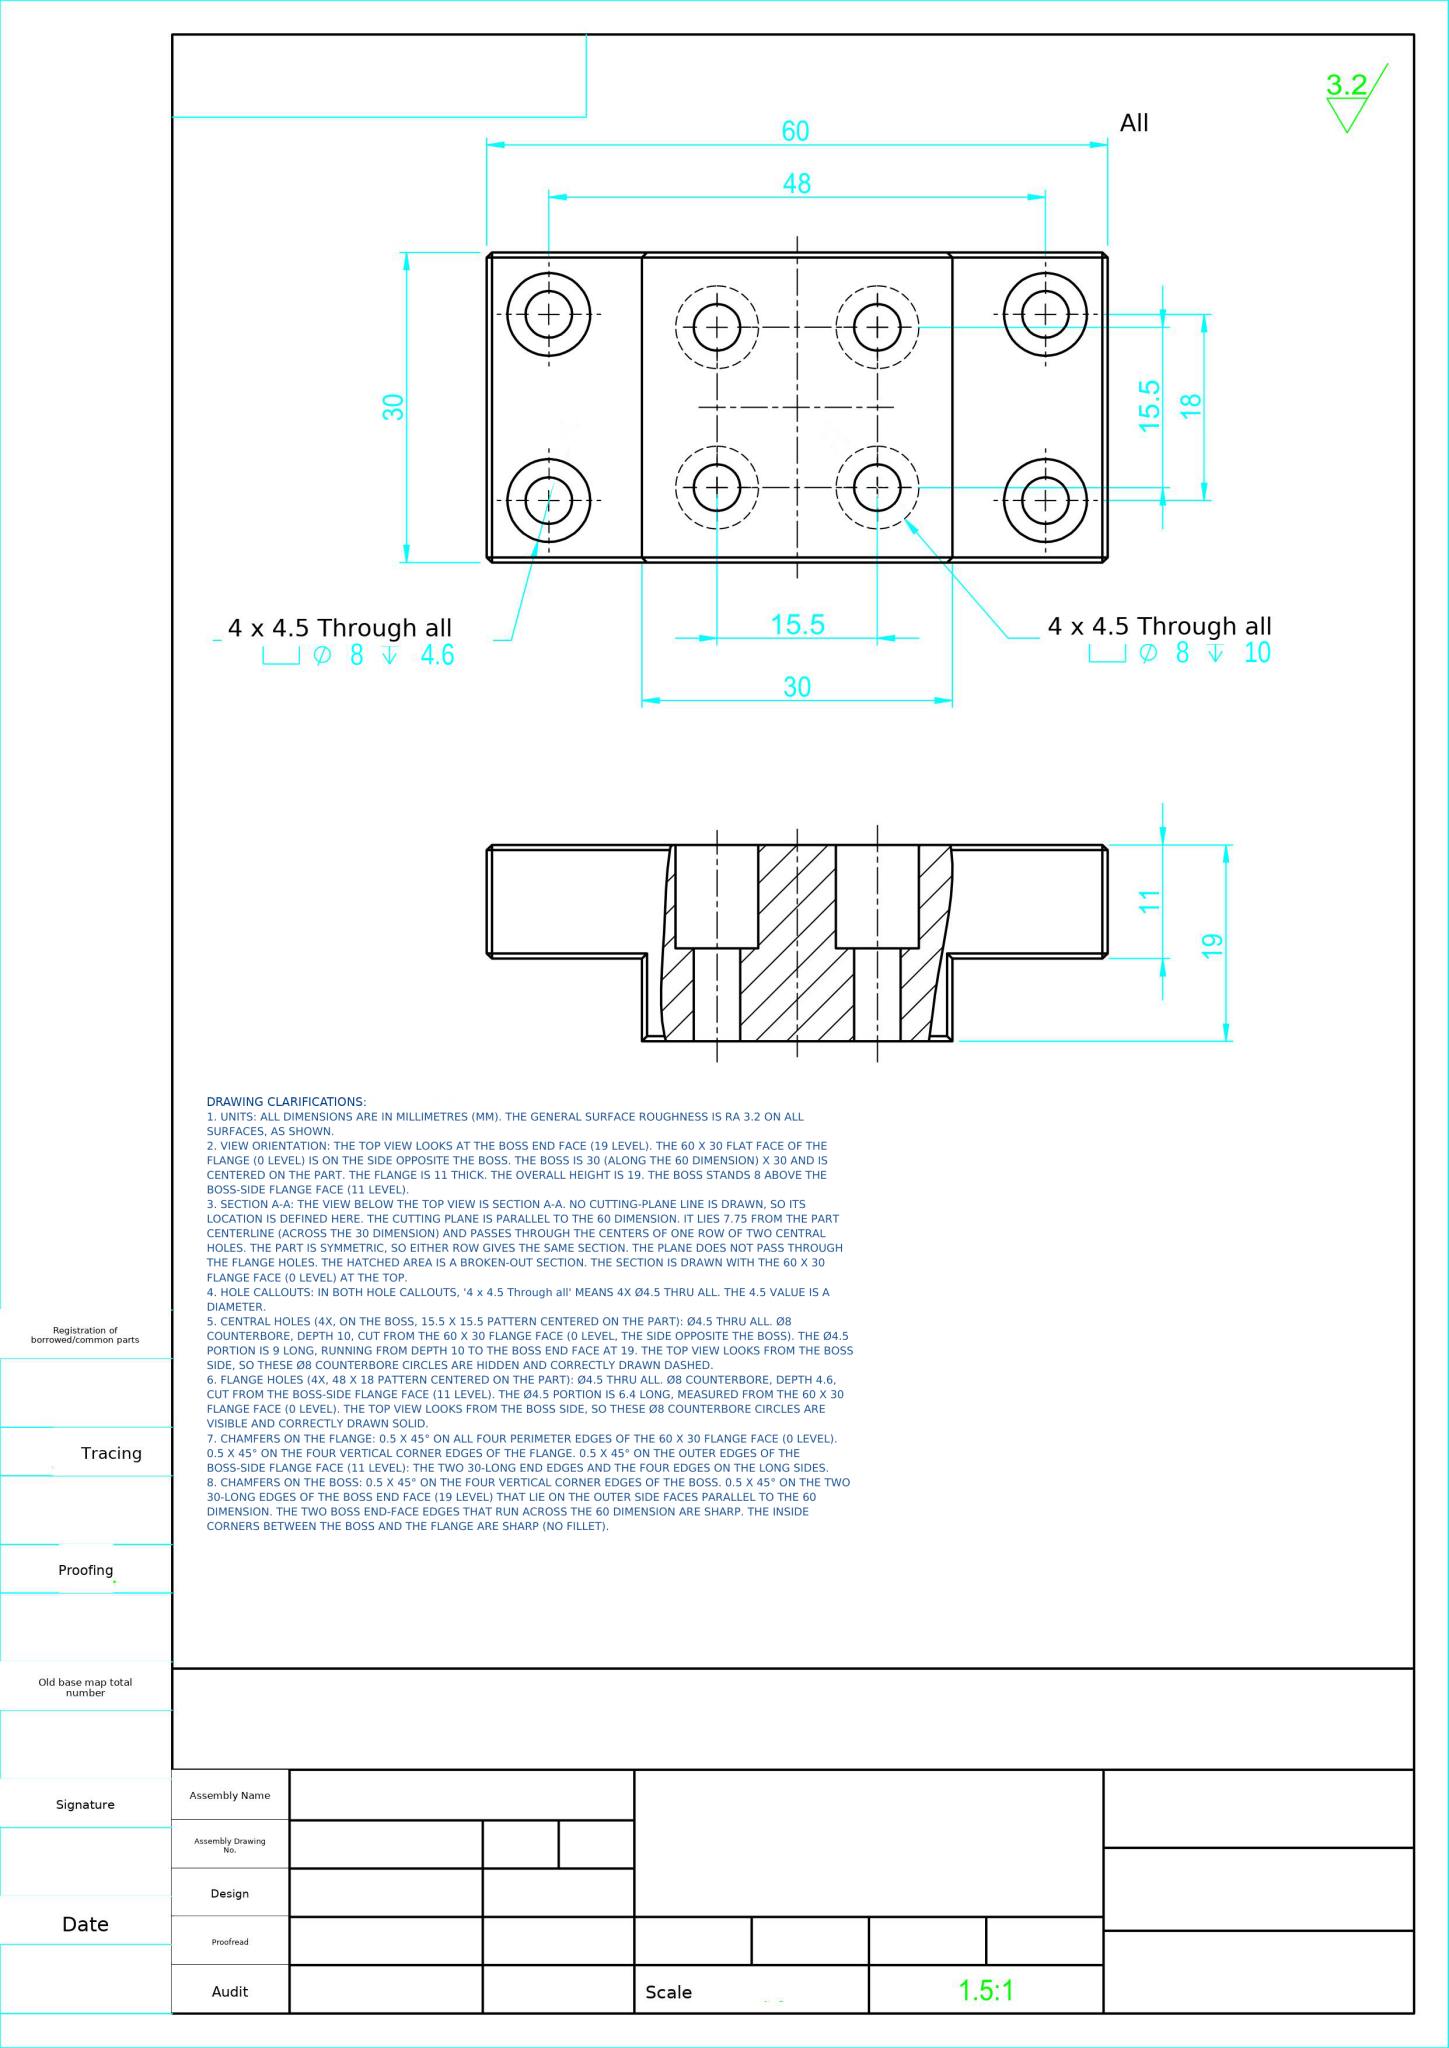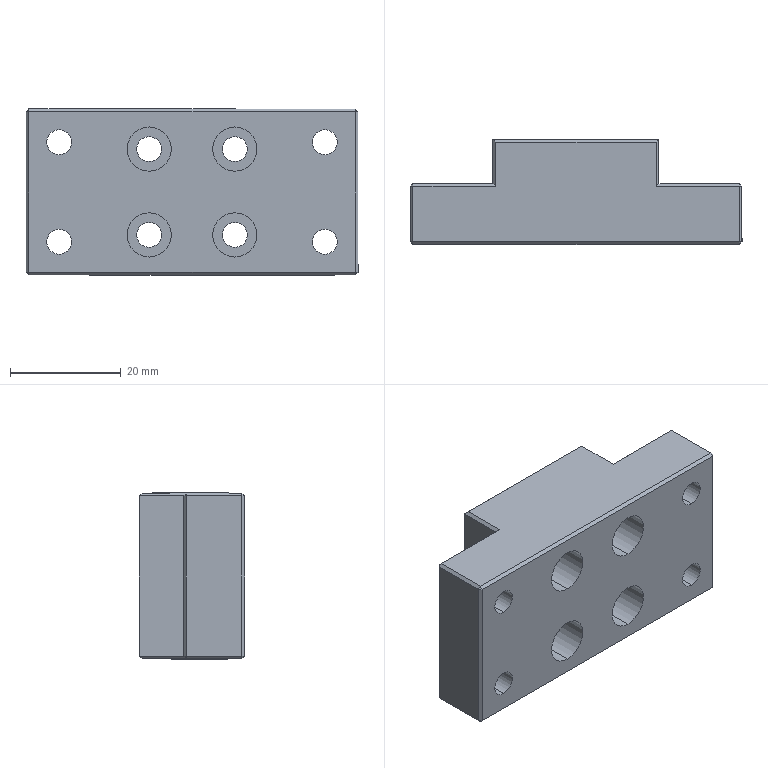Part | NX | mm | 1 solid | 78 faces | box 60 x 19 x 30 mm | volume 23031 mm3 | plane 46 | cylinder 32 | commonest cylinder face diameters 8 x16 4.5 x16